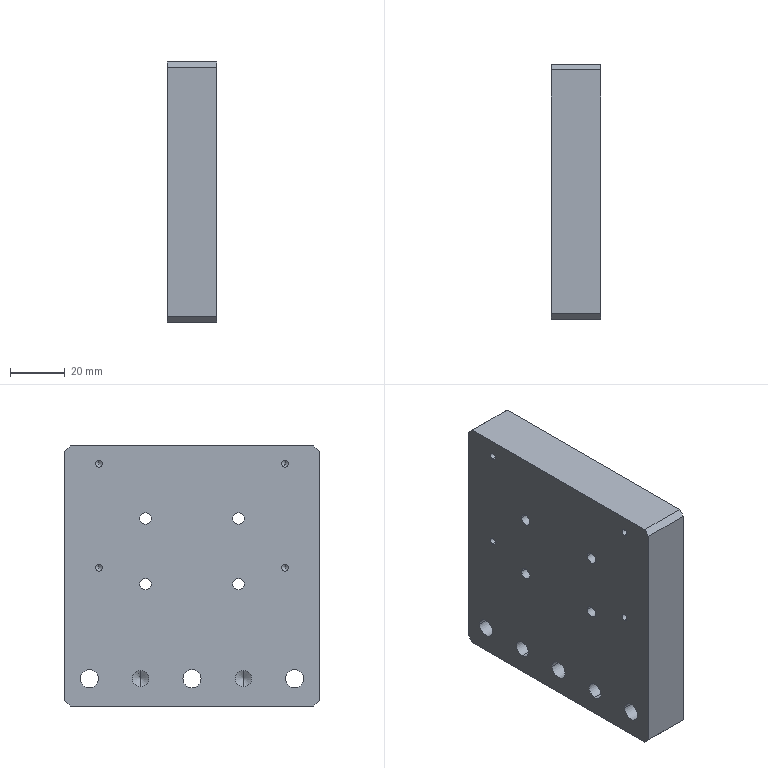Component | SolidWorks | AX.B92.SA.7371.25-2 | 1 solid | 57 faces | box 18 x 93 x 95 mm | volume 154049 mm3 | cylinder 32 | plane 13 | cone 12 | commonest cylinder face diameters 2.5 x8 4.2 x8 11 x6 6.6 x6 6 x4 | material 7075
build123d program:
from build123d import *

# Parameters (mm, degrees)
SKETCH1_W                                          = 18
SKETCH1_H                                          = 95
BOSS_EXTRUDE1_DEPTH                                = 46.5
M5_TAPPED_HOLE1_D                                  = 4.2
CHAMFER1_SIZE                                      = 2
HOLE_SIZE_ACCORDING_TO_TYPE_1_OF_HEXAG_D           = 6.6
HOLE_SIZE_ACCORDING_TO_TYPE_1_OF_HEXAG_CBORE_D     = 11
HOLE_SIZE_ACCORDING_TO_TYPE_1_OF_HEXAG_CBORE_DEPTH = 6.8
SIZE_MM_DOWEL_PIN_HOLE1_D                          = 6
SIZE_MM_DOWEL_PIN_HOLE1_DEPTH                      = 10
SIZE_MM_DOWEL_PIN_HOLE1_TIP                        = 1.803
M3_TAPPED_HOLE1_D                                  = 2.5
M3_TAPPED_HOLE1_DEPTH                              = 7.5
M3_TAPPED_HOLE1_TIP                                = 0.7511


with BuildPart() as part:
    # Sketch1 → Boss-Extrude1 (new, symmetric)
    with BuildSketch(Plane(origin=(0, 0, 0), x_dir=(0, 0, -1), z_dir=(1, 0, 0))):
        Rectangle(SKETCH1_W, SKETCH1_H)
    extrude(amount=BOSS_EXTRUDE1_DEPTH, both=True)

    # M5 Tapped Hole1 (through all)
    with Locations(Plane.XY.offset(9)):
        with Locations((-17, -21), (-17, 3), (17, 3), (17, -21)):
            Hole(M5_TAPPED_HOLE1_D / 2)

    # Chamfer1
    chamfer1_edges = [part.edges().sort_by_distance(p)[0] for p in [
        (46.5, -47.5, 0),
        (46.5, 47.5, 0),
        (-46.5, -47.5, 0),
        (-46.5, 47.5, 0),
    ]]
    chamfer(chamfer1_edges, length=CHAMFER1_SIZE)

    # Hole Size _according to_ Type 1 of Hexag (through all)
    with Locations(Plane.XY.offset(9)):
        with Locations((-37.5, 37.5), (0, 37.5), (37.5, 37.5)):
            CounterBoreHole(HOLE_SIZE_ACCORDING_TO_TYPE_1_OF_HEXAG_D / 2, HOLE_SIZE_ACCORDING_TO_TYPE_1_OF_HEXAG_CBORE_D / 2, HOLE_SIZE_ACCORDING_TO_TYPE_1_OF_HEXAG_CBORE_DEPTH)

    # Size mm Dowel Pin Hole1
    with Locations(Plane(origin=(0, 0, -9), x_dir=(-1, 0, 0), z_dir=(0, 0, -1))):
        with Locations((-18.75, 37.5), (18.75, 37.5)):
            Hole(SIZE_MM_DOWEL_PIN_HOLE1_D / 2, depth=SIZE_MM_DOWEL_PIN_HOLE1_DEPTH)
            with Locations((0, 0, -(SIZE_MM_DOWEL_PIN_HOLE1_DEPTH + SIZE_MM_DOWEL_PIN_HOLE1_TIP / 2))):  # 118° drill point
                Cone(0, SIZE_MM_DOWEL_PIN_HOLE1_D / 2, SIZE_MM_DOWEL_PIN_HOLE1_TIP, mode=Mode.SUBTRACT)

    # M3 Tapped Hole1
    with Locations(Plane(origin=(0, 0, -9), x_dir=(-1, 0, 0), z_dir=(0, 0, -1))):
        with Locations((-34, -3), (-34, -41), (34, -3), (34, -41)):
            Hole(M3_TAPPED_HOLE1_D / 2, depth=M3_TAPPED_HOLE1_DEPTH)
            with Locations((0, 0, -(M3_TAPPED_HOLE1_DEPTH + M3_TAPPED_HOLE1_TIP / 2))):  # 118° drill point
                Cone(0, M3_TAPPED_HOLE1_D / 2, M3_TAPPED_HOLE1_TIP, mode=Mode.SUBTRACT)


solid = part.part

# Placed as in the assembly
solid = solid.moved(Location((-9.579, 53.688, 75.972), (-90, 90, 0)))